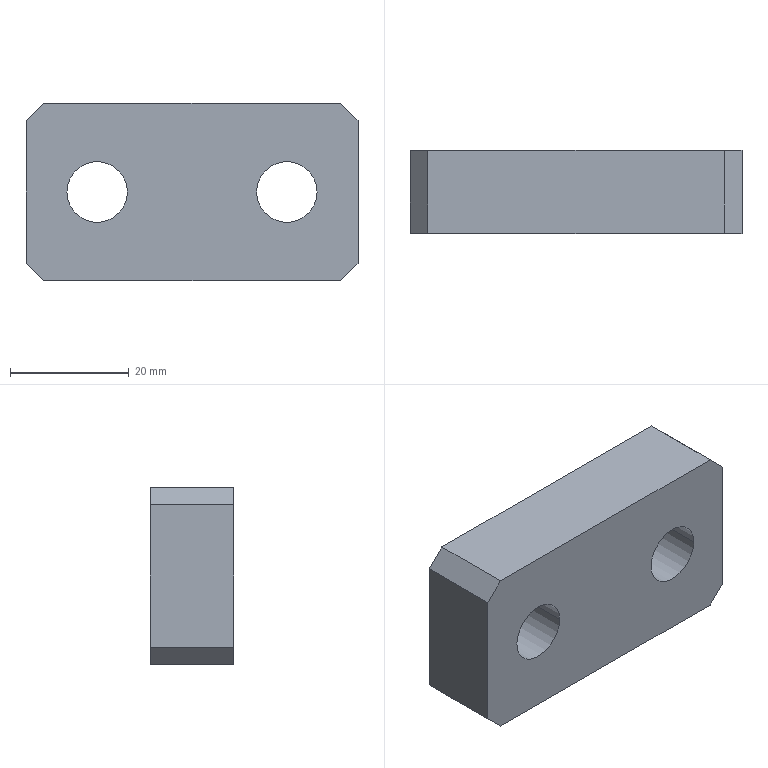Component | SolidWorks | PressurePlateFixingSeat-2 | 1 solid | 14 faces | box 56 x 14 x 30 mm | volume 20980 mm3 | plane 10 | cylinder 4 | commonest cylinder face diameters 10.2 x4
build123d program:
from build123d import *

# Parameters (mm, degrees)
SKETCH1_W              = 56
SKETCH1_H              = 30
BOSS_EXTRUDE1_DEPTH    = 14
M12_TAPPED_HOLE1_D     = 10.2
M12_TAPPED_HOLE1_DEPTH = 29.25
M12_TAPPED_HOLE1_TIP   = 3.064
CHAMFER1_SIZE          = 3


with BuildPart() as part:
    # Sketch1 → Boss-Extrude1 (new body)
    with BuildSketch(Plane.XY):
        Rectangle(SKETCH1_W, SKETCH1_H)
    extrude(amount=BOSS_EXTRUDE1_DEPTH)

    # M12 Tapped Hole1
    with Locations(Plane(origin=(-16, 0, 14), x_dir=(1, 0, 0), z_dir=(0, 0, 1))):
        with Locations((0, 0), (32, 0)):
            Hole(M12_TAPPED_HOLE1_D / 2, depth=M12_TAPPED_HOLE1_DEPTH)
            with Locations((0, 0, -(M12_TAPPED_HOLE1_DEPTH + M12_TAPPED_HOLE1_TIP / 2))):  # 118° drill point
                Cone(0, M12_TAPPED_HOLE1_D / 2, M12_TAPPED_HOLE1_TIP, mode=Mode.SUBTRACT)

    # Chamfer1
    chamfer1_edges = [part.edges().sort_by_distance(p)[0] for p in [
        (28, -15, 7),
        (-28, -15, 7),
        (-28, 15, 7),
        (28, 15, 7),
    ]]
    chamfer(chamfer1_edges, length=CHAMFER1_SIZE)


solid = part.part

# Placed as in the assembly
solid = solid.moved(Location((-112, 179.606, 0), (90, 0, 0)))
STEP:
#1=COLOUR_RGB('',0.7922,0.8196,0.9333);
#2=FILL_AREA_STYLE_COLOUR('',#1);
#3=FILL_AREA_STYLE('',(#2));
#4=SURFACE_STYLE_FILL_AREA(#3);
#5=SURFACE_SIDE_STYLE('',(#4));
#6=SURFACE_STYLE_USAGE(.BOTH.,#5);
#7=PRESENTATION_STYLE_ASSIGNMENT((#6));
#8=CARTESIAN_POINT('',(-3.98,7.071,0.));
#9=VERTEX_POINT('',#8);
#10=CARTESIAN_POINT('',(-3.579,7.071,-0.));
#11=VERTEX_POINT('',#10);
#12=CARTESIAN_POINT('',(-3.78,7.071,0.));
#13=DIRECTION('',(0.,1.,0.));
#14=DIRECTION('',(1.,0.,0.));
#15=AXIS2_PLACEMENT_3D('',#12,#13,#14);
#16=CIRCLE('',#15,0.2008);
#17=EDGE_CURVE('',#9,#11,#16,.T.);
#18=ORIENTED_EDGE('',*,*,#17,.T.);
#19=CARTESIAN_POINT('',(-3.579,6.52,-0.));
#20=VERTEX_POINT('',#19);
#21=CARTESIAN_POINT('',(-3.579,6.52,-0.));
#22=DIRECTION('',(0.,-1.,0.));
#23=VECTOR('',#22,39.37);
#24=LINE('',#21,#23);
#25=EDGE_CURVE('',#11,#20,#24,.T.);
#26=ORIENTED_EDGE('',*,*,#25,.T.);
#27=CARTESIAN_POINT('',(-3.98,6.52,0.));
#28=VERTEX_POINT('',#27);
#29=CARTESIAN_POINT('',(-3.78,6.52,0.));
#30=DIRECTION('',(0.,-1.,0.));
#31=DIRECTION('',(-1.,0.,0.));
#32=AXIS2_PLACEMENT_3D('',#29,#30,#31);
#33=CIRCLE('',#32,0.2008);
#34=EDGE_CURVE('',#20,#28,#33,.T.);
#35=ORIENTED_EDGE('',*,*,#34,.T.);
#36=CARTESIAN_POINT('',(-3.98,6.52,0.));
#37=DIRECTION('',(0.,-1.,0.));
#38=VECTOR('',#37,39.37);
#39=LINE('',#36,#38);
#40=EDGE_CURVE('',#9,#28,#39,.T.);
#41=ORIENTED_EDGE('',*,*,#40,.F.);
#42=EDGE_LOOP('',(#18,#26,#35,#41));
#43=FACE_OUTER_BOUND('',#42,.T.);
#44=CARTESIAN_POINT('',(-3.78,6.52,0.));
#45=DIRECTION('',(0.,-1.,0.));
#46=DIRECTION('',(-1.,0.,0.));
#47=AXIS2_PLACEMENT_3D('',#44,#45,#46);
#48=CYLINDRICAL_SURFACE('',#47,0.2008);
#49=ADVANCED_FACE('',(#43),#48,.F.);
#50=CARTESIAN_POINT('',(-5.24,7.071,0.));
#51=VERTEX_POINT('',#50);
#52=CARTESIAN_POINT('',(-4.839,7.071,-0.));
#53=VERTEX_POINT('',#52);
#54=CARTESIAN_POINT('',(-5.039,7.071,0.));
#55=DIRECTION('',(0.,1.,0.));
#56=DIRECTION('',(1.,0.,0.));
#57=AXIS2_PLACEMENT_3D('',#54,#55,#56);
#58=CIRCLE('',#57,0.2008);
#59=EDGE_CURVE('',#51,#53,#58,.T.);
#60=ORIENTED_EDGE('',*,*,#59,.T.);
#61=CARTESIAN_POINT('',(-4.839,6.52,-0.));
#62=VERTEX_POINT('',#61);
#63=CARTESIAN_POINT('',(-4.839,6.52,-0.));
#64=DIRECTION('',(0.,-1.,0.));
#65=VECTOR('',#64,39.37);
#66=LINE('',#63,#65);
#67=EDGE_CURVE('',#53,#62,#66,.T.);
#68=ORIENTED_EDGE('',*,*,#67,.T.);
#69=CARTESIAN_POINT('',(-5.24,6.52,0.));
#70=VERTEX_POINT('',#69);
#71=CARTESIAN_POINT('',(-5.039,6.52,0.));
#72=DIRECTION('',(0.,-1.,0.));
#73=DIRECTION('',(-1.,0.,0.));
#74=AXIS2_PLACEMENT_3D('',#71,#72,#73);
#75=CIRCLE('',#74,0.2008);
#76=EDGE_CURVE('',#62,#70,#75,.T.);
#77=ORIENTED_EDGE('',*,*,#76,.T.);
#78=CARTESIAN_POINT('',(-5.24,6.52,0.));
#79=DIRECTION('',(0.,-1.,0.));
#80=VECTOR('',#79,39.37);
#81=LINE('',#78,#80);
#82=EDGE_CURVE('',#51,#70,#81,.T.);
#83=ORIENTED_EDGE('',*,*,#82,.F.);
#84=EDGE_LOOP('',(#60,#68,#77,#83));
#85=FACE_OUTER_BOUND('',#84,.T.);
#86=CARTESIAN_POINT('',(-5.039,6.52,0.));
#87=DIRECTION('',(0.,-1.,0.));
#88=DIRECTION('',(-1.,0.,0.));
#89=AXIS2_PLACEMENT_3D('',#86,#87,#88);
#90=CYLINDRICAL_SURFACE('',#89,0.2008);
#91=ADVANCED_FACE('',(#85),#90,.F.);
#92=CARTESIAN_POINT('',(-5.512,6.52,0.4724));
#93=VERTEX_POINT('',#92);
#94=CARTESIAN_POINT('',(-5.512,6.52,-0.4724));
#95=VERTEX_POINT('',#94);
#96=CARTESIAN_POINT('',(-5.512,6.52,0.5906));
#97=DIRECTION('',(0.,0.,-1.));
#98=VECTOR('',#97,39.37);
#99=LINE('',#96,#98);
#100=EDGE_CURVE('',#93,#95,#99,.T.);
#101=ORIENTED_EDGE('',*,*,#100,.F.);
#102=CARTESIAN_POINT('',(-5.512,7.071,0.4724));
#103=VERTEX_POINT('',#102);
#104=CARTESIAN_POINT('',(-5.512,6.52,0.4724));
#105=DIRECTION('',(0.,1.,0.));
#106=VECTOR('',#105,39.37);
#107=LINE('',#104,#106);
#108=EDGE_CURVE('',#93,#103,#107,.T.);
#109=ORIENTED_EDGE('',*,*,#108,.T.);
#110=CARTESIAN_POINT('',(-5.512,7.071,-0.4724));
#111=VERTEX_POINT('',#110);
#112=CARTESIAN_POINT('',(-5.512,7.071,0.5906));
#113=DIRECTION('',(0.,0.,-1.));
#114=VECTOR('',#113,39.37);
#115=LINE('',#112,#114);
#116=EDGE_CURVE('',#103,#111,#115,.T.);
#117=ORIENTED_EDGE('',*,*,#116,.T.);
#118=CARTESIAN_POINT('',(-5.512,6.52,-0.4724));
#119=DIRECTION('',(0.,-1.,0.));
#120=VECTOR('',#119,39.37);
#121=LINE('',#118,#120);
#122=EDGE_CURVE('',#111,#95,#121,.T.);
#123=ORIENTED_EDGE('',*,*,#122,.T.);
#124=EDGE_LOOP('',(#101,#109,#117,#123));
#125=FACE_OUTER_BOUND('',#124,.T.);
#126=CARTESIAN_POINT('',(-5.512,6.52,0.5906));
#127=DIRECTION('',(1.,0.,0.));
#128=DIRECTION('',(0.,-1.,0.));
#129=AXIS2_PLACEMENT_3D('',#126,#127,#128);
#130=PLANE('',#129);
#131=ADVANCED_FACE('',(#125),#130,.F.);
#132=CARTESIAN_POINT('',(-5.394,7.071,-0.5906));
#133=VERTEX_POINT('',#132);
#134=CARTESIAN_POINT('',(-3.425,7.071,-0.5906));
#135=VERTEX_POINT('',#134);
#136=CARTESIAN_POINT('',(-3.307,7.071,-0.5906));
#137=DIRECTION('',(1.,0.,0.));
#138=VECTOR('',#137,39.37);
#139=LINE('',#136,#138);
#140=EDGE_CURVE('',#133,#135,#139,.T.);
#141=ORIENTED_EDGE('',*,*,#140,.T.);
#142=CARTESIAN_POINT('',(-3.425,6.52,-0.5906));
#143=VERTEX_POINT('',#142);
#144=CARTESIAN_POINT('',(-3.425,6.52,-0.5906));
#145=DIRECTION('',(0.,-1.,0.));
#146=VECTOR('',#145,39.37);
#147=LINE('',#144,#146);
#148=EDGE_CURVE('',#135,#143,#147,.T.);
#149=ORIENTED_EDGE('',*,*,#148,.T.);
#150=CARTESIAN_POINT('',(-5.394,6.52,-0.5906));
#151=VERTEX_POINT('',#150);
#152=CARTESIAN_POINT('',(-3.307,6.52,-0.5906));
#153=DIRECTION('',(1.,0.,0.));
#154=VECTOR('',#153,39.37);
#155=LINE('',#152,#154);
#156=EDGE_CURVE('',#151,#143,#155,.T.);
#157=ORIENTED_EDGE('',*,*,#156,.F.);
#158=CARTESIAN_POINT('',(-5.394,6.52,-0.5906));
#159=DIRECTION('',(0.,1.,0.));
#160=VECTOR('',#159,39.37);
#161=LINE('',#158,#160);
#162=EDGE_CURVE('',#151,#133,#161,.T.);
#163=ORIENTED_EDGE('',*,*,#162,.T.);
#164=EDGE_LOOP('',(#141,#149,#157,#163));
#165=FACE_OUTER_BOUND('',#164,.T.);
#166=CARTESIAN_POINT('',(-3.307,6.52,-0.5906));
#167=DIRECTION('',(0.,0.,1.));
#168=DIRECTION('',(0.,1.,0.));
#169=AXIS2_PLACEMENT_3D('',#166,#167,#168);
#170=PLANE('',#169);
#171=ADVANCED_FACE('',(#165),#170,.F.);
#172=CARTESIAN_POINT('',(-3.307,6.52,-0.4724));
#173=VERTEX_POINT('',#172);
#174=CARTESIAN_POINT('',(-3.307,6.52,0.4724));
#175=VERTEX_POINT('',#174);
#176=CARTESIAN_POINT('',(-3.307,6.52,0.5906));
#177=DIRECTION('',(0.,0.,1.));
#178=VECTOR('',#177,39.37);
#179=LINE('',#176,#178);
#180=EDGE_CURVE('',#173,#175,#179,.T.);
#181=ORIENTED_EDGE('',*,*,#180,.F.);
#182=CARTESIAN_POINT('',(-3.307,7.071,-0.4724));
#183=VERTEX_POINT('',#182);
#184=CARTESIAN_POINT('',(-3.307,6.52,-0.4724));
#185=DIRECTION('',(0.,1.,0.));
#186=VECTOR('',#185,39.37);
#187=LINE('',#184,#186);
#188=EDGE_CURVE('',#173,#183,#187,.T.);
#189=ORIENTED_EDGE('',*,*,#188,.T.);
#190=CARTESIAN_POINT('',(-3.307,7.071,0.4724));
#191=VERTEX_POINT('',#190);
#192=CARTESIAN_POINT('',(-3.307,7.071,0.5906));
#193=DIRECTION('',(0.,0.,1.));
#194=VECTOR('',#193,39.37);
#195=LINE('',#192,#194);
#196=EDGE_CURVE('',#183,#191,#195,.T.);
#197=ORIENTED_EDGE('',*,*,#196,.T.);
#198=CARTESIAN_POINT('',(-3.307,6.52,0.4724));
#199=DIRECTION('',(0.,-1.,0.));
#200=VECTOR('',#199,39.37);
#201=LINE('',#198,#200);
#202=EDGE_CURVE('',#191,#175,#201,.T.);
#203=ORIENTED_EDGE('',*,*,#202,.T.);
#204=EDGE_LOOP('',(#181,#189,#197,#203));
#205=FACE_OUTER_BOUND('',#204,.T.);
#206=CARTESIAN_POINT('',(-3.307,6.52,0.5906));
#207=DIRECTION('',(-1.,0.,0.));
#208=DIRECTION('',(0.,1.,0.));
#209=AXIS2_PLACEMENT_3D('',#206,#207,#208);
#210=PLANE('',#209);
#211=ADVANCED_FACE('',(#205),#210,.F.);
#212=CARTESIAN_POINT('',(-3.425,6.52,0.5906));
#213=VERTEX_POINT('',#212);
#214=CARTESIAN_POINT('',(-5.394,6.52,0.5906));
#215=VERTEX_POINT('',#214);
#216=CARTESIAN_POINT('',(-3.307,6.52,0.5906));
#217=DIRECTION('',(-1.,0.,0.));
#218=VECTOR('',#217,39.37);
#219=LINE('',#216,#218);
#220=EDGE_CURVE('',#213,#215,#219,.T.);
#221=ORIENTED_EDGE('',*,*,#220,.F.);
#222=CARTESIAN_POINT('',(-3.425,7.071,0.5906));
#223=VERTEX_POINT('',#222);
#224=CARTESIAN_POINT('',(-3.425,6.52,0.5906));
#225=DIRECTION('',(0.,1.,0.));
#226=VECTOR('',#225,39.37);
#227=LINE('',#224,#226);
#228=EDGE_CURVE('',#213,#223,#227,.T.);
#229=ORIENTED_EDGE('',*,*,#228,.T.);
#230=CARTESIAN_POINT('',(-5.394,7.071,0.5906));
#231=VERTEX_POINT('',#230);
#232=CARTESIAN_POINT('',(-3.307,7.071,0.5906));
#233=DIRECTION('',(-1.,0.,0.));
#234=VECTOR('',#233,39.37);
#235=LINE('',#232,#234);
#236=EDGE_CURVE('',#223,#231,#235,.T.);
#237=ORIENTED_EDGE('',*,*,#236,.T.);
#238=CARTESIAN_POINT('',(-5.394,6.52,0.5906));
#239=DIRECTION('',(0.,-1.,0.));
#240=VECTOR('',#239,39.37);
#241=LINE('',#238,#240);
#242=EDGE_CURVE('',#231,#215,#241,.T.);
#243=ORIENTED_EDGE('',*,*,#242,.T.);
#244=EDGE_LOOP('',(#221,#229,#237,#243));
#245=FACE_OUTER_BOUND('',#244,.T.);
#246=CARTESIAN_POINT('',(-3.307,6.52,0.5906));
#247=DIRECTION('',(0.,0.,-1.));
#248=DIRECTION('',(0.,-1.,0.));
#249=AXIS2_PLACEMENT_3D('',#246,#247,#248);
#250=PLANE('',#249);
#251=ADVANCED_FACE('',(#245),#250,.F.);
#252=CARTESIAN_POINT('',(-3.78,6.52,0.));
#253=DIRECTION('',(0.,-1.,0.));
#254=DIRECTION('',(-1.,0.,0.));
#255=AXIS2_PLACEMENT_3D('',#252,#253,#254);
#256=CIRCLE('',#255,0.2008);
#257=EDGE_CURVE('',#28,#20,#256,.T.);
#258=ORIENTED_EDGE('',*,*,#257,.F.);
#259=ORIENTED_EDGE('',*,*,#34,.F.);
#260=EDGE_LOOP('',(#258,#259));
#261=FACE_BOUND('',#260,.T.);
#262=CARTESIAN_POINT('',(-5.039,6.52,0.));
#263=DIRECTION('',(0.,-1.,0.));
#264=DIRECTION('',(-1.,0.,0.));
#265=AXIS2_PLACEMENT_3D('',#262,#263,#264);
#266=CIRCLE('',#265,0.2008);
#267=EDGE_CURVE('',#70,#62,#266,.T.);
#268=ORIENTED_EDGE('',*,*,#267,.F.);
#269=ORIENTED_EDGE('',*,*,#76,.F.);
#270=EDGE_LOOP('',(#268,#269));
#271=FACE_BOUND('',#270,.T.);
#272=ORIENTED_EDGE('',*,*,#156,.T.);
#273=CARTESIAN_POINT('',(-3.307,6.52,-0.4724));
#274=DIRECTION('',(0.7071,0.,0.7071));
#275=VECTOR('',#274,39.37);
#276=LINE('',#273,#275);
#277=EDGE_CURVE('',#143,#173,#276,.T.);
#278=ORIENTED_EDGE('',*,*,#277,.T.);
#279=ORIENTED_EDGE('',*,*,#180,.T.);
#280=CARTESIAN_POINT('',(-3.425,6.52,0.5906));
#281=DIRECTION('',(-0.7071,0.,0.7071));
#282=VECTOR('',#281,39.37);
#283=LINE('',#280,#282);
#284=EDGE_CURVE('',#175,#213,#283,.T.);
#285=ORIENTED_EDGE('',*,*,#284,.T.);
#286=ORIENTED_EDGE('',*,*,#220,.T.);
#287=CARTESIAN_POINT('',(-5.512,6.52,0.4724));
#288=DIRECTION('',(-0.7071,0.,-0.7071));
#289=VECTOR('',#288,39.37);
#290=LINE('',#287,#289);
#291=EDGE_CURVE('',#215,#93,#290,.T.);
#292=ORIENTED_EDGE('',*,*,#291,.T.);
#293=ORIENTED_EDGE('',*,*,#100,.T.);
#294=CARTESIAN_POINT('',(-5.394,6.52,-0.5906));
#295=DIRECTION('',(0.7071,0.,-0.7071));
#296=VECTOR('',#295,39.37);
#297=LINE('',#294,#296);
#298=EDGE_CURVE('',#95,#151,#297,.T.);
#299=ORIENTED_EDGE('',*,*,#298,.T.);
#300=EDGE_LOOP('',(#272,#278,#279,#285,#286,#292,#293,#299));
#301=FACE_OUTER_BOUND('',#300,.T.);
#302=CARTESIAN_POINT('',(-4.409,6.52,0.));
#303=DIRECTION('',(0.,1.,0.));
#304=DIRECTION('',(1.,0.,0.));
#305=AXIS2_PLACEMENT_3D('',#302,#303,#304);
#306=PLANE('',#305);
#307=ADVANCED_FACE('',(#261,#271,#301),#306,.F.);
#308=ORIENTED_EDGE('',*,*,#17,.F.);
#309=CARTESIAN_POINT('',(-3.78,7.071,0.));
#310=DIRECTION('',(0.,1.,0.));
#311=DIRECTION('',(1.,0.,0.));
#312=AXIS2_PLACEMENT_3D('',#309,#310,#311);
#313=CIRCLE('',#312,0.2008);
#314=EDGE_CURVE('',#11,#9,#313,.T.);
#315=ORIENTED_EDGE('',*,*,#314,.F.);
#316=EDGE_LOOP('',(#308,#315));
#317=FACE_BOUND('',#316,.T.);
#318=ORIENTED_EDGE('',*,*,#59,.F.);
#319=CARTESIAN_POINT('',(-5.039,7.071,0.));
#320=DIRECTION('',(0.,1.,0.));
#321=DIRECTION('',(1.,0.,0.));
#322=AXIS2_PLACEMENT_3D('',#319,#320,#321);
#323=CIRCLE('',#322,0.2008);
#324=EDGE_CURVE('',#53,#51,#323,.T.);
#325=ORIENTED_EDGE('',*,*,#324,.F.);
#326=EDGE_LOOP('',(#318,#325));
#327=FACE_BOUND('',#326,.T.);
#328=ORIENTED_EDGE('',*,*,#196,.F.);
#329=CARTESIAN_POINT('',(-3.622,7.071,-0.7874));
#330=DIRECTION('',(-0.7071,0.,-0.7071));
#331=VECTOR('',#330,39.37);
#332=LINE('',#329,#331);
#333=EDGE_CURVE('',#183,#135,#332,.T.);
#334=ORIENTED_EDGE('',*,*,#333,.T.);
#335=ORIENTED_EDGE('',*,*,#140,.F.);
#336=CARTESIAN_POINT('',(-5.197,7.071,-0.7874));
#337=DIRECTION('',(-0.7071,0.,0.7071));
#338=VECTOR('',#337,39.37);
#339=LINE('',#336,#338);
#340=EDGE_CURVE('',#133,#111,#339,.T.);
#341=ORIENTED_EDGE('',*,*,#340,.T.);
#342=ORIENTED_EDGE('',*,*,#116,.F.);
#343=CARTESIAN_POINT('',(-5.197,7.071,0.7874));
#344=DIRECTION('',(0.7071,0.,0.7071));
#345=VECTOR('',#344,39.37);
#346=LINE('',#343,#345);
#347=EDGE_CURVE('',#103,#231,#346,.T.);
#348=ORIENTED_EDGE('',*,*,#347,.T.);
#349=ORIENTED_EDGE('',*,*,#236,.F.);
#350=CARTESIAN_POINT('',(-3.622,7.071,0.7874));
#351=DIRECTION('',(0.7071,0.,-0.7071));
#352=VECTOR('',#351,39.37);
#353=LINE('',#350,#352);
#354=EDGE_CURVE('',#223,#191,#353,.T.);
#355=ORIENTED_EDGE('',*,*,#354,.T.);
#356=EDGE_LOOP('',(#328,#334,#335,#341,#342,#348,#349,#355));
#357=FACE_OUTER_BOUND('',#356,.T.);
#358=CARTESIAN_POINT('',(-4.409,7.071,0.));
#359=DIRECTION('',(0.,1.,0.));
#360=DIRECTION('',(1.,0.,0.));
#361=AXIS2_PLACEMENT_3D('',#358,#359,#360);
#362=PLANE('',#361);
#363=ADVANCED_FACE('',(#317,#327,#357),#362,.T.);
#364=ORIENTED_EDGE('',*,*,#67,.F.);
#365=ORIENTED_EDGE('',*,*,#324,.T.);
#366=ORIENTED_EDGE('',*,*,#82,.T.);
#367=ORIENTED_EDGE('',*,*,#267,.T.);
#368=EDGE_LOOP('',(#364,#365,#366,#367));
#369=FACE_OUTER_BOUND('',#368,.T.);
#370=CARTESIAN_POINT('',(-5.039,6.52,0.));
#371=DIRECTION('',(0.,-1.,0.));
#372=DIRECTION('',(-1.,0.,0.));
#373=AXIS2_PLACEMENT_3D('',#370,#371,#372);
#374=CYLINDRICAL_SURFACE('',#373,0.2008);
#375=ADVANCED_FACE('',(#369),#374,.F.);
#376=ORIENTED_EDGE('',*,*,#25,.F.);
#377=ORIENTED_EDGE('',*,*,#314,.T.);
#378=ORIENTED_EDGE('',*,*,#40,.T.);
#379=ORIENTED_EDGE('',*,*,#257,.T.);
#380=EDGE_LOOP('',(#376,#377,#378,#379));
#381=FACE_OUTER_BOUND('',#380,.T.);
#382=CARTESIAN_POINT('',(-3.78,6.52,0.));
#383=DIRECTION('',(0.,-1.,0.));
#384=DIRECTION('',(-1.,0.,0.));
#385=AXIS2_PLACEMENT_3D('',#382,#383,#384);
#386=CYLINDRICAL_SURFACE('',#385,0.2008);
#387=ADVANCED_FACE('',(#381),#386,.F.);
#388=ORIENTED_EDGE('',*,*,#277,.F.);
#389=ORIENTED_EDGE('',*,*,#148,.F.);
#390=ORIENTED_EDGE('',*,*,#333,.F.);
#391=ORIENTED_EDGE('',*,*,#188,.F.);
#392=EDGE_LOOP('',(#388,#389,#390,#391));
#393=FACE_OUTER_BOUND('',#392,.T.);
#394=CARTESIAN_POINT('',(-3.307,6.52,-0.4724));
#395=DIRECTION('',(-0.7071,0.,0.7071));
#396=DIRECTION('',(0.,1.,0.));
#397=AXIS2_PLACEMENT_3D('',#394,#395,#396);
#398=PLANE('',#397);
#399=ADVANCED_FACE('',(#393),#398,.F.);
#400=ORIENTED_EDGE('',*,*,#284,.F.);
#401=ORIENTED_EDGE('',*,*,#202,.F.);
#402=ORIENTED_EDGE('',*,*,#354,.F.);
#403=ORIENTED_EDGE('',*,*,#228,.F.);
#404=EDGE_LOOP('',(#400,#401,#402,#403));
#405=FACE_OUTER_BOUND('',#404,.T.);
#406=CARTESIAN_POINT('',(-3.425,6.52,0.5906));
#407=DIRECTION('',(-0.7071,0.,-0.7071));
#408=DIRECTION('',(0.,1.,0.));
#409=AXIS2_PLACEMENT_3D('',#406,#407,#408);
#410=PLANE('',#409);
#411=ADVANCED_FACE('',(#405),#410,.F.);
#412=ORIENTED_EDGE('',*,*,#291,.F.);
#413=ORIENTED_EDGE('',*,*,#242,.F.);
#414=ORIENTED_EDGE('',*,*,#347,.F.);
#415=ORIENTED_EDGE('',*,*,#108,.F.);
#416=EDGE_LOOP('',(#412,#413,#414,#415));
#417=FACE_OUTER_BOUND('',#416,.T.);
#418=CARTESIAN_POINT('',(-5.512,6.52,0.4724));
#419=DIRECTION('',(0.7071,0.,-0.7071));
#420=DIRECTION('',(0.,1.,0.));
#421=AXIS2_PLACEMENT_3D('',#418,#419,#420);
#422=PLANE('',#421);
#423=ADVANCED_FACE('',(#417),#422,.F.);
#424=ORIENTED_EDGE('',*,*,#298,.F.);
#425=ORIENTED_EDGE('',*,*,#122,.F.);
#426=ORIENTED_EDGE('',*,*,#340,.F.);
#427=ORIENTED_EDGE('',*,*,#162,.F.);
#428=EDGE_LOOP('',(#424,#425,#426,#427));
#429=FACE_OUTER_BOUND('',#428,.T.);
#430=CARTESIAN_POINT('',(-5.394,6.52,-0.5906));
#431=DIRECTION('',(0.7071,0.,0.7071));
#432=DIRECTION('',(0.,1.,0.));
#433=AXIS2_PLACEMENT_3D('',#430,#431,#432);
#434=PLANE('',#433);
#435=ADVANCED_FACE('',(#429),#434,.F.);
#436=CLOSED_SHELL('',(#49,#91,#131,#171,#211,#251,#307,#363,#375,#387,#399,#411,#423,#435));
#437=MANIFOLD_SOLID_BREP('',#436);
#438=STYLED_ITEM('',(#7),#437);
#439=PRESENTATION_LAYER_ASSIGNMENT('','',(#438));
#440=CARTESIAN_POINT('',(0.,0.,0.));
#441=DIRECTION('',(0.,0.,1.));
#442=DIRECTION('',(1.,0.,0.));
#443=AXIS2_PLACEMENT_3D('',#440,#441,#442);
#444=(LENGTH_UNIT()NAMED_UNIT(*)SI_UNIT($,.METRE.));
#445=LENGTH_MEASURE_WITH_UNIT(LENGTH_MEASURE(0.0254),#444);
#446=DIMENSIONAL_EXPONENTS(1.,0.,0.,0.,0.,0.,0.);
#447=(CONVERSION_BASED_UNIT('',#445)LENGTH_UNIT()NAMED_UNIT(#446));
#448=UNCERTAINTY_MEASURE_WITH_UNIT(LENGTH_MEASURE(0.00001),#447,'','');
#449=(NAMED_UNIT(*)PLANE_ANGLE_UNIT()SI_UNIT($,.RADIAN.));
#450=(NAMED_UNIT(*)SI_UNIT($,.STERADIAN.)SOLID_ANGLE_UNIT());
#451=(GEOMETRIC_REPRESENTATION_CONTEXT(3)GLOBAL_UNCERTAINTY_ASSIGNED_CONTEXT((#448))GLOBAL_UNIT_ASSIGNED_CONTEXT((#447,#449,#450))REPRESENTATION_CONTEXT('',''));
#452=ADVANCED_BREP_SHAPE_REPRESENTATION('',(#437,#443),#451);
#453=(LENGTH_UNIT()NAMED_UNIT(*)SI_UNIT($,.METRE.));
#454=LENGTH_MEASURE_WITH_UNIT(LENGTH_MEASURE(0.0254),#453);
#455=DIMENSIONAL_EXPONENTS(1.,0.,0.,0.,0.,0.,0.);
#456=(CONVERSION_BASED_UNIT('',#454)LENGTH_UNIT()NAMED_UNIT(#455));
#457=UNCERTAINTY_MEASURE_WITH_UNIT(LENGTH_MEASURE(0.00001),#456,'','');
#458=(NAMED_UNIT(*)PLANE_ANGLE_UNIT()SI_UNIT($,.RADIAN.));
#459=(NAMED_UNIT(*)SI_UNIT($,.STERADIAN.)SOLID_ANGLE_UNIT());
#460=(GEOMETRIC_REPRESENTATION_CONTEXT(3)GLOBAL_UNCERTAINTY_ASSIGNED_CONTEXT((#457))GLOBAL_UNIT_ASSIGNED_CONTEXT((#456,#458,#459))REPRESENTATION_CONTEXT('',''));
#461=MECHANICAL_DESIGN_GEOMETRIC_PRESENTATION_REPRESENTATION('',(#438),#460);